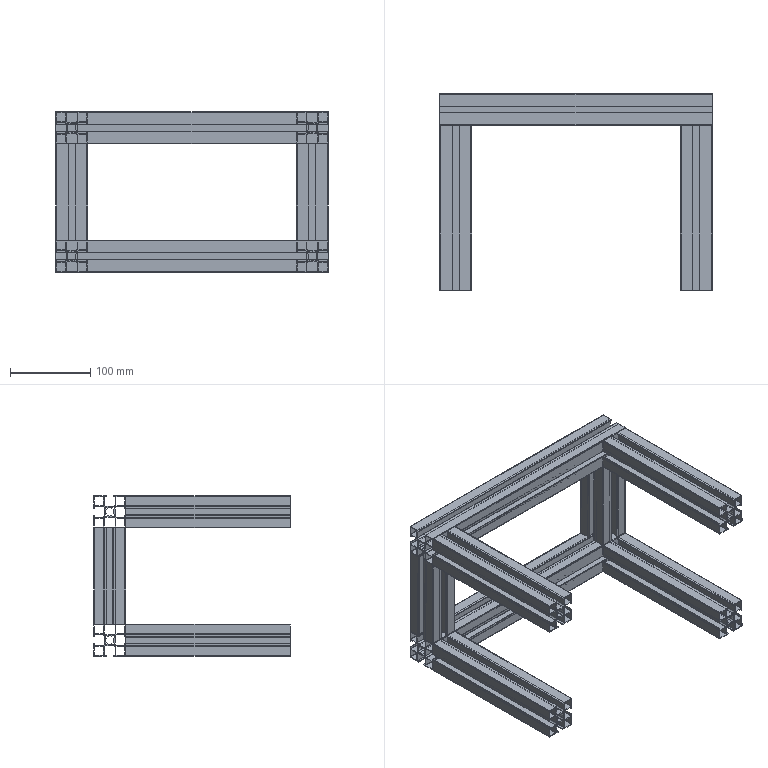Component | SolidWorks | LH-CGJ-01-056-1 | 8 solids | 680 faces | volume 515658 mm3 | plane 496 | cylinder 184 | commonest cylinder face diameters 4 x64 2.8 x48 10.4 x40 2 x32 | material SKD11